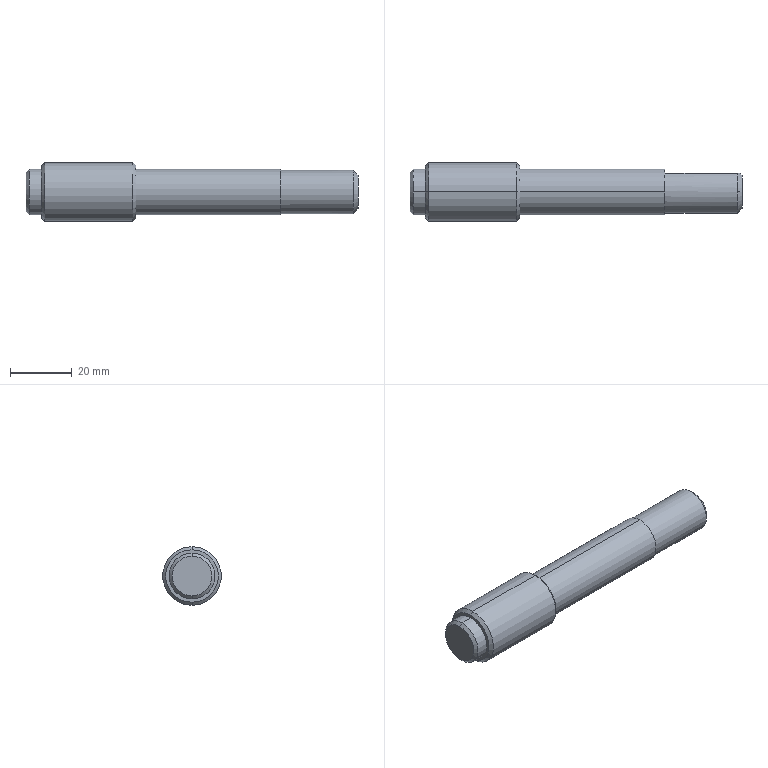CAM job | Mastercam | mm | 2 operations | part box 107.6 x 19 x 19
1. Contour (2D) | 21 - 12 平铣刀
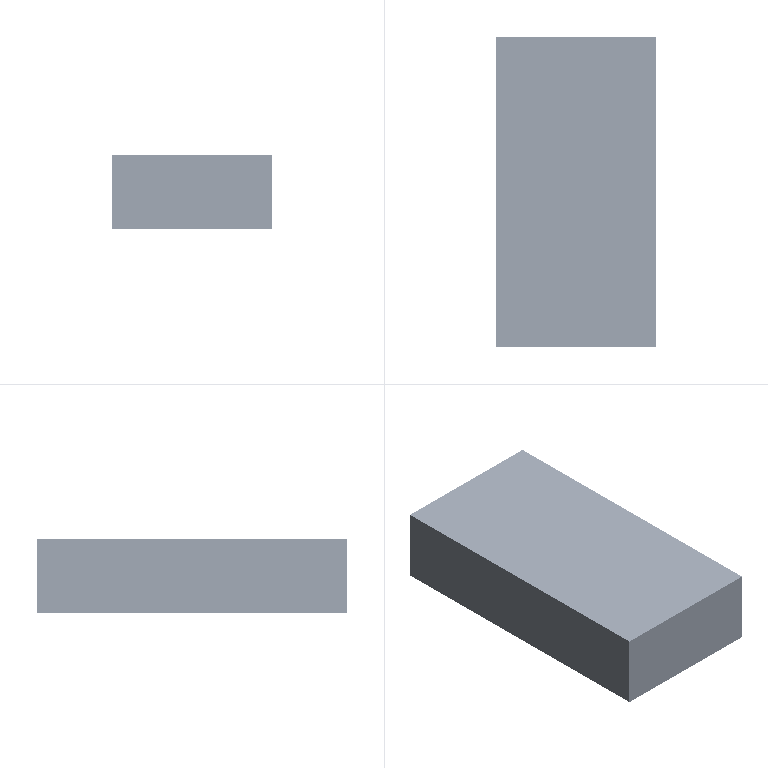2. Drill/Counterbore | 5 - 4 倒角刀